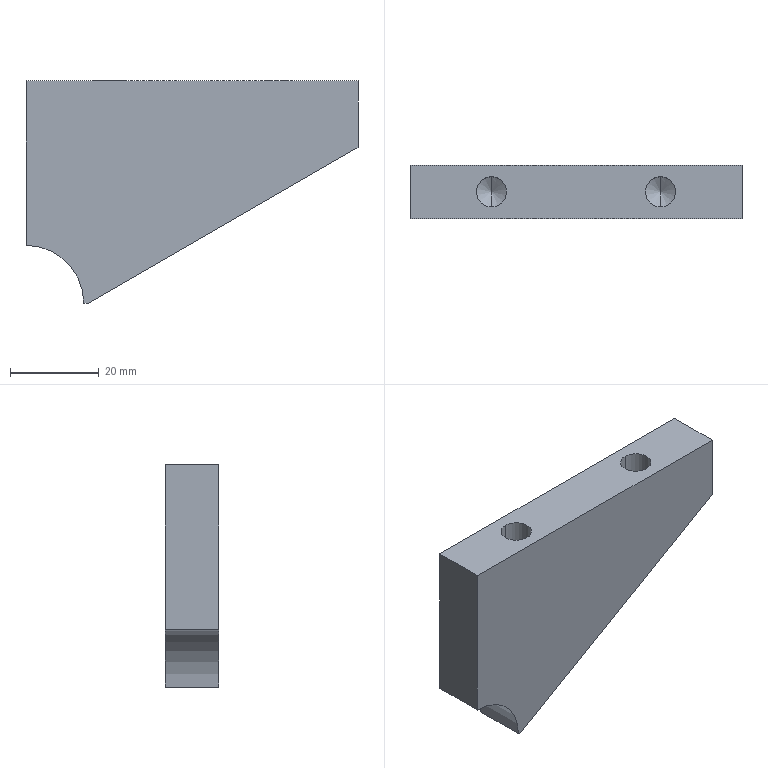Component | SolidWorks | StopBlock2-1 | 1 solid | 16 faces | box 74.62 x 12 x 50 mm | volume 28966 mm3 | plane 7 | cylinder 5 | cone 4 | commonest cylinder face diameters 6.8 x4 26 x1 | material Q235
build123d program:
from build123d import *

# Parameters (mm, degrees)
BOSS_EXTRUDE1_DEPTH   = 12
M8_TAPPED_HOLE1_D     = 6.8
M8_TAPPED_HOLE1_DEPTH = 19.75
M8_TAPPED_HOLE1_TIP   = 2.043
SKETCH4_R             = 13
CUT_EXTRUDE1_DEPTH    = 91.622


with BuildPart() as part:
    # Sketch1 → Boss-Extrude1 (new body)
    with BuildSketch(Plane.XY):
        Polygon((0, 0), (0, 50), (-14, 50), (-74.622, 15), (-74.622, 0), align=None)
    extrude(amount=BOSS_EXTRUDE1_DEPTH)

    # M8 Tapped Hole1
    with Locations(Plane(origin=(-56.311, 0, 6), x_dir=(0, 0, -1), z_dir=(0, -1, 0))):
        with Locations((0, 0), (0, 38)):
            Hole(M8_TAPPED_HOLE1_D / 2, depth=M8_TAPPED_HOLE1_DEPTH)
            with Locations((0, 0, -(M8_TAPPED_HOLE1_DEPTH + M8_TAPPED_HOLE1_TIP / 2))):  # 118° drill point
                Cone(0, M8_TAPPED_HOLE1_D / 2, M8_TAPPED_HOLE1_TIP, mode=Mode.SUBTRACT)

    # Sketch4 → Cut-Extrude1 (cut, through all)
    with BuildSketch(Plane.XY.offset(12)):
        with Locations((0, 50)):
            Circle(SKETCH4_R)
    extrude(amount=-CUT_EXTRUDE1_DEPTH, mode=Mode.SUBTRACT)


solid = part.part

# Placed as in the assembly
solid = solid.moved(Location((1.474, -118.917, -1190.957), (90, 0, -180)))
STEP:
#1=COLOUR_RGB('',0.7922,0.8196,0.9333);
#2=FILL_AREA_STYLE_COLOUR('',#1);
#3=FILL_AREA_STYLE('',(#2));
#4=SURFACE_STYLE_FILL_AREA(#3);
#5=SURFACE_SIDE_STYLE('',(#4));
#6=SURFACE_STYLE_USAGE(.BOTH.,#5);
#7=PRESENTATION_STYLE_ASSIGNMENT((#6));
#8=CARTESIAN_POINT('',(2.275,-5.052,-47.666));
#9=VERTEX_POINT('',#8);
#10=CARTESIAN_POINT('',(2.275,-4.784,-47.666));
#11=VERTEX_POINT('',#10);
#12=CARTESIAN_POINT('',(2.275,-4.918,-47.666));
#13=DIRECTION('',(0.,0.,1.));
#14=DIRECTION('',(0.,1.,0.));
#15=AXIS2_PLACEMENT_3D('',#12,#13,#14);
#16=CIRCLE('',#15,0.1339);
#17=EDGE_CURVE('',#9,#11,#16,.T.);
#18=ORIENTED_EDGE('',*,*,#17,.F.);
#19=CARTESIAN_POINT('',(2.275,-5.052,-46.888));
#20=VERTEX_POINT('',#19);
#21=CARTESIAN_POINT('',(2.275,-5.052,-46.888));
#22=DIRECTION('',(0.,0.,1.));
#23=VECTOR('',#22,39.37);
#24=LINE('',#21,#23);
#25=EDGE_CURVE('',#9,#20,#24,.T.);
#26=ORIENTED_EDGE('',*,*,#25,.T.);
#27=CARTESIAN_POINT('',(2.275,-4.784,-46.888));
#28=VERTEX_POINT('',#27);
#29=CARTESIAN_POINT('',(2.275,-4.918,-46.888));
#30=DIRECTION('',(0.,0.,1.));
#31=DIRECTION('',(0.,1.,0.));
#32=AXIS2_PLACEMENT_3D('',#29,#30,#31);
#33=CIRCLE('',#32,0.1339);
#34=EDGE_CURVE('',#20,#28,#33,.T.);
#35=ORIENTED_EDGE('',*,*,#34,.T.);
#36=CARTESIAN_POINT('',(2.275,-4.784,-46.888));
#37=DIRECTION('',(0.,0.,1.));
#38=VECTOR('',#37,39.37);
#39=LINE('',#36,#38);
#40=EDGE_CURVE('',#11,#28,#39,.T.);
#41=ORIENTED_EDGE('',*,*,#40,.F.);
#42=EDGE_LOOP('',(#18,#26,#35,#41));
#43=FACE_OUTER_BOUND('',#42,.T.);
#44=CARTESIAN_POINT('',(2.275,-4.918,-46.888));
#45=DIRECTION('',(0.,0.,1.));
#46=DIRECTION('',(0.,1.,0.));
#47=AXIS2_PLACEMENT_3D('',#44,#45,#46);
#48=CYLINDRICAL_SURFACE('',#47,0.1339);
#49=ADVANCED_FACE('',(#43),#48,.F.);
#50=CARTESIAN_POINT('',(2.275,-4.918,-47.746));
#51=VERTEX_POINT('',#50);
#52=CARTESIAN_POINT('',(2.275,-4.784,-47.666));
#53=DIRECTION('',(0.,0.8572,0.515));
#54=VECTOR('',#53,39.37);
#55=LINE('',#52,#54);
#56=EDGE_CURVE('',#51,#11,#55,.T.);
#57=ORIENTED_EDGE('',*,*,#56,.F.);
#58=CARTESIAN_POINT('',(2.275,-5.052,-47.666));
#59=DIRECTION('',(-0.,-0.8572,0.515));
#60=VECTOR('',#59,39.37);
#61=LINE('',#58,#60);
#62=EDGE_CURVE('',#51,#9,#61,.T.);
#63=ORIENTED_EDGE('',*,*,#62,.T.);
#64=ORIENTED_EDGE('',*,*,#17,.T.);
#65=EDGE_LOOP('',(#57,#63,#64));
#66=FACE_OUTER_BOUND('',#65,.T.);
#67=CARTESIAN_POINT('',(2.275,-4.918,-47.666));
#68=DIRECTION('',(0.,0.,1.));
#69=DIRECTION('',(0.,1.,0.));
#70=AXIS2_PLACEMENT_3D('',#67,#68,#69);
#71=CONICAL_SURFACE('',#70,0.1339,1.03);
#72=ADVANCED_FACE('',(#66),#71,.F.);
#73=CARTESIAN_POINT('',(0.7789,-5.052,-47.666));
#74=VERTEX_POINT('',#73);
#75=CARTESIAN_POINT('',(0.7789,-4.784,-47.666));
#76=VERTEX_POINT('',#75);
#77=CARTESIAN_POINT('',(0.7789,-4.918,-47.666));
#78=DIRECTION('',(0.,0.,1.));
#79=DIRECTION('',(0.,1.,0.));
#80=AXIS2_PLACEMENT_3D('',#77,#78,#79);
#81=CIRCLE('',#80,0.1339);
#82=EDGE_CURVE('',#74,#76,#81,.T.);
#83=ORIENTED_EDGE('',*,*,#82,.F.);
#84=CARTESIAN_POINT('',(0.7789,-5.052,-46.888));
#85=VERTEX_POINT('',#84);
#86=CARTESIAN_POINT('',(0.7789,-5.052,-46.888));
#87=DIRECTION('',(0.,0.,1.));
#88=VECTOR('',#87,39.37);
#89=LINE('',#86,#88);
#90=EDGE_CURVE('',#74,#85,#89,.T.);
#91=ORIENTED_EDGE('',*,*,#90,.T.);
#92=CARTESIAN_POINT('',(0.7789,-4.784,-46.888));
#93=VERTEX_POINT('',#92);
#94=CARTESIAN_POINT('',(0.7789,-4.918,-46.888));
#95=DIRECTION('',(0.,0.,1.));
#96=DIRECTION('',(0.,1.,0.));
#97=AXIS2_PLACEMENT_3D('',#94,#95,#96);
#98=CIRCLE('',#97,0.1339);
#99=EDGE_CURVE('',#85,#93,#98,.T.);
#100=ORIENTED_EDGE('',*,*,#99,.T.);
#101=CARTESIAN_POINT('',(0.7789,-4.784,-46.888));
#102=DIRECTION('',(0.,0.,1.));
#103=VECTOR('',#102,39.37);
#104=LINE('',#101,#103);
#105=EDGE_CURVE('',#76,#93,#104,.T.);
#106=ORIENTED_EDGE('',*,*,#105,.F.);
#107=EDGE_LOOP('',(#83,#91,#100,#106));
#108=FACE_OUTER_BOUND('',#107,.T.);
#109=CARTESIAN_POINT('',(0.7789,-4.918,-46.888));
#110=DIRECTION('',(0.,0.,1.));
#111=DIRECTION('',(0.,1.,0.));
#112=AXIS2_PLACEMENT_3D('',#109,#110,#111);
#113=CYLINDRICAL_SURFACE('',#112,0.1339);
#114=ADVANCED_FACE('',(#108),#113,.F.);
#115=CARTESIAN_POINT('',(0.7789,-4.918,-47.746));
#116=VERTEX_POINT('',#115);
#117=CARTESIAN_POINT('',(0.7789,-4.784,-47.666));
#118=DIRECTION('',(0.,0.8572,0.515));
#119=VECTOR('',#118,39.37);
#120=LINE('',#117,#119);
#121=EDGE_CURVE('',#116,#76,#120,.T.);
#122=ORIENTED_EDGE('',*,*,#121,.F.);
#123=CARTESIAN_POINT('',(0.7789,-5.052,-47.666));
#124=DIRECTION('',(-0.,-0.8572,0.515));
#125=VECTOR('',#124,39.37);
#126=LINE('',#123,#125);
#127=EDGE_CURVE('',#116,#74,#126,.T.);
#128=ORIENTED_EDGE('',*,*,#127,.T.);
#129=ORIENTED_EDGE('',*,*,#82,.T.);
#130=EDGE_LOOP('',(#122,#128,#129));
#131=FACE_OUTER_BOUND('',#130,.T.);
#132=CARTESIAN_POINT('',(0.7789,-4.918,-47.666));
#133=DIRECTION('',(0.,0.,1.));
#134=DIRECTION('',(0.,1.,0.));
#135=AXIS2_PLACEMENT_3D('',#132,#133,#134);
#136=CONICAL_SURFACE('',#135,0.1339,1.03);
#137=ADVANCED_FACE('',(#131),#136,.F.);
#138=CARTESIAN_POINT('',(2.275,-4.918,-46.888));
#139=DIRECTION('',(0.,0.,1.));
#140=DIRECTION('',(0.,1.,0.));
#141=AXIS2_PLACEMENT_3D('',#138,#139,#140);
#142=CIRCLE('',#141,0.1339);
#143=EDGE_CURVE('',#28,#20,#142,.T.);
#144=ORIENTED_EDGE('',*,*,#143,.F.);
#145=ORIENTED_EDGE('',*,*,#34,.F.);
#146=EDGE_LOOP('',(#144,#145));
#147=FACE_BOUND('',#146,.T.);
#148=CARTESIAN_POINT('',(0.7789,-4.918,-46.888));
#149=DIRECTION('',(0.,0.,1.));
#150=DIRECTION('',(0.,1.,0.));
#151=AXIS2_PLACEMENT_3D('',#148,#149,#150);
#152=CIRCLE('',#151,0.1339);
#153=EDGE_CURVE('',#93,#85,#152,.T.);
#154=ORIENTED_EDGE('',*,*,#153,.F.);
#155=ORIENTED_EDGE('',*,*,#99,.F.);
#156=EDGE_LOOP('',(#154,#155));
#157=FACE_BOUND('',#156,.T.);
#158=CARTESIAN_POINT('',(2.996,-4.682,-46.888));
#159=VERTEX_POINT('',#158);
#160=CARTESIAN_POINT('',(0.05803,-4.682,-46.888));
#161=VERTEX_POINT('',#160);
#162=CARTESIAN_POINT('',(2.996,-4.682,-46.888));
#163=DIRECTION('',(-1.,0.,0.));
#164=VECTOR('',#163,39.37);
#165=LINE('',#162,#164);
#166=EDGE_CURVE('',#159,#161,#165,.T.);
#167=ORIENTED_EDGE('',*,*,#166,.T.);
#168=CARTESIAN_POINT('',(0.05803,-5.154,-46.888));
#169=VERTEX_POINT('',#168);
#170=CARTESIAN_POINT('',(0.05803,-5.154,-46.888));
#171=DIRECTION('',(0.,1.,0.));
#172=VECTOR('',#171,39.37);
#173=LINE('',#170,#172);
#174=EDGE_CURVE('',#169,#161,#173,.T.);
#175=ORIENTED_EDGE('',*,*,#174,.F.);
#176=CARTESIAN_POINT('',(2.996,-5.154,-46.888));
#177=VERTEX_POINT('',#176);
#178=CARTESIAN_POINT('',(2.996,-5.154,-46.888));
#179=DIRECTION('',(-1.,0.,0.));
#180=VECTOR('',#179,39.37);
#181=LINE('',#178,#180);
#182=EDGE_CURVE('',#177,#169,#181,.T.);
#183=ORIENTED_EDGE('',*,*,#182,.F.);
#184=CARTESIAN_POINT('',(2.996,-5.154,-46.888));
#185=DIRECTION('',(0.,1.,0.));
#186=VECTOR('',#185,39.37);
#187=LINE('',#184,#186);
#188=EDGE_CURVE('',#177,#159,#187,.T.);
#189=ORIENTED_EDGE('',*,*,#188,.T.);
#190=EDGE_LOOP('',(#167,#175,#183,#189));
#191=FACE_OUTER_BOUND('',#190,.T.);
#192=CARTESIAN_POINT('',(2.996,-5.154,-46.888));
#193=DIRECTION('',(0.,0.,-1.));
#194=DIRECTION('',(0.,-1.,0.));
#195=AXIS2_PLACEMENT_3D('',#192,#193,#194);
#196=PLANE('',#195);
#197=ADVANCED_FACE('',(#147,#157,#191),#196,.F.);
#198=CARTESIAN_POINT('',(0.05803,-4.682,-48.345));
#199=VERTEX_POINT('',#198);
#200=CARTESIAN_POINT('',(0.05803,-4.682,-46.888));
#201=DIRECTION('',(0.,0.,-1.));
#202=VECTOR('',#201,39.37);
#203=LINE('',#200,#202);
#204=EDGE_CURVE('',#161,#199,#203,.T.);
#205=ORIENTED_EDGE('',*,*,#204,.T.);
#206=CARTESIAN_POINT('',(0.05803,-5.154,-48.345));
#207=VERTEX_POINT('',#206);
#208=CARTESIAN_POINT('',(0.05803,-4.682,-48.345));
#209=DIRECTION('',(0.,-1.,0.));
#210=VECTOR('',#209,39.37);
#211=LINE('',#208,#210);
#212=EDGE_CURVE('',#199,#207,#211,.T.);
#213=ORIENTED_EDGE('',*,*,#212,.T.);
#214=CARTESIAN_POINT('',(0.05803,-5.154,-46.888));
#215=DIRECTION('',(0.,0.,-1.));
#216=VECTOR('',#215,39.37);
#217=LINE('',#214,#216);
#218=EDGE_CURVE('',#169,#207,#217,.T.);
#219=ORIENTED_EDGE('',*,*,#218,.F.);
#220=ORIENTED_EDGE('',*,*,#174,.T.);
#221=EDGE_LOOP('',(#205,#213,#219,#220));
#222=FACE_OUTER_BOUND('',#221,.T.);
#223=CARTESIAN_POINT('',(0.05803,-5.154,-46.888));
#224=DIRECTION('',(1.,0.,0.));
#225=DIRECTION('',(0.,-1.,0.));
#226=AXIS2_PLACEMENT_3D('',#223,#224,#225);
#227=PLANE('',#226);
#228=ADVANCED_FACE('',(#222),#227,.F.);
#229=CARTESIAN_POINT('',(0.5698,-5.154,-48.857));
#230=VERTEX_POINT('',#229);
#231=CARTESIAN_POINT('',(0.6092,-5.154,-48.857));
#232=VERTEX_POINT('',#231);
#233=CARTESIAN_POINT('',(0.05803,-5.154,-48.857));
#234=DIRECTION('',(1.,0.,0.));
#235=VECTOR('',#234,39.37);
#236=LINE('',#233,#235);
#237=EDGE_CURVE('',#230,#232,#236,.T.);
#238=ORIENTED_EDGE('',*,*,#237,.F.);
#239=CARTESIAN_POINT('',(0.5698,-4.682,-48.857));
#240=VERTEX_POINT('',#239);
#241=CARTESIAN_POINT('',(0.5698,-4.682,-48.857));
#242=DIRECTION('',(0.,1.,0.));
#243=VECTOR('',#242,39.37);
#244=LINE('',#241,#243);
#245=EDGE_CURVE('',#230,#240,#244,.T.);
#246=ORIENTED_EDGE('',*,*,#245,.T.);
#247=CARTESIAN_POINT('',(0.6092,-4.682,-48.857));
#248=VERTEX_POINT('',#247);
#249=CARTESIAN_POINT('',(0.05803,-4.682,-48.857));
#250=DIRECTION('',(1.,0.,0.));
#251=VECTOR('',#250,39.37);
#252=LINE('',#249,#251);
#253=EDGE_CURVE('',#240,#248,#252,.T.);
#254=ORIENTED_EDGE('',*,*,#253,.T.);
#255=CARTESIAN_POINT('',(0.6092,-5.154,-48.857));
#256=DIRECTION('',(0.,1.,0.));
#257=VECTOR('',#256,39.37);
#258=LINE('',#255,#257);
#259=EDGE_CURVE('',#232,#248,#258,.T.);
#260=ORIENTED_EDGE('',*,*,#259,.F.);
#261=EDGE_LOOP('',(#238,#246,#254,#260));
#262=FACE_OUTER_BOUND('',#261,.T.);
#263=CARTESIAN_POINT('',(0.05803,-5.154,-48.857));
#264=DIRECTION('',(0.,0.,1.));
#265=DIRECTION('',(0.,1.,0.));
#266=AXIS2_PLACEMENT_3D('',#263,#264,#265);
#267=PLANE('',#266);
#268=ADVANCED_FACE('',(#262),#267,.F.);
#269=CARTESIAN_POINT('',(2.996,-4.682,-47.479));
#270=VERTEX_POINT('',#269);
#271=CARTESIAN_POINT('',(2.996,-4.682,-47.479));
#272=DIRECTION('',(0.866,0.,0.5));
#273=VECTOR('',#272,39.37);
#274=LINE('',#271,#273);
#275=EDGE_CURVE('',#248,#270,#274,.T.);
#276=ORIENTED_EDGE('',*,*,#275,.T.);
#277=CARTESIAN_POINT('',(2.996,-5.154,-47.479));
#278=VERTEX_POINT('',#277);
#279=CARTESIAN_POINT('',(2.996,-5.154,-47.479));
#280=DIRECTION('',(0.,1.,0.));
#281=VECTOR('',#280,39.37);
#282=LINE('',#279,#281);
#283=EDGE_CURVE('',#278,#270,#282,.T.);
#284=ORIENTED_EDGE('',*,*,#283,.F.);
#285=CARTESIAN_POINT('',(2.996,-5.154,-47.479));
#286=DIRECTION('',(0.866,0.,0.5));
#287=VECTOR('',#286,39.37);
#288=LINE('',#285,#287);
#289=EDGE_CURVE('',#232,#278,#288,.T.);
#290=ORIENTED_EDGE('',*,*,#289,.F.);
#291=ORIENTED_EDGE('',*,*,#259,.T.);
#292=EDGE_LOOP('',(#276,#284,#290,#291));
#293=FACE_OUTER_BOUND('',#292,.T.);
#294=CARTESIAN_POINT('',(2.996,-5.154,-47.479));
#295=DIRECTION('',(-0.5,0.,0.866));
#296=DIRECTION('',(-0.866,0.,-0.5));
#297=AXIS2_PLACEMENT_3D('',#294,#295,#296);
#298=PLANE('',#297);
#299=ADVANCED_FACE('',(#293),#298,.F.);
#300=CARTESIAN_POINT('',(2.996,-4.682,-46.888));
#301=DIRECTION('',(0.,0.,1.));
#302=VECTOR('',#301,39.37);
#303=LINE('',#300,#302);
#304=EDGE_CURVE('',#270,#159,#303,.T.);
#305=ORIENTED_EDGE('',*,*,#304,.T.);
#306=ORIENTED_EDGE('',*,*,#188,.F.);
#307=CARTESIAN_POINT('',(2.996,-5.154,-46.888));
#308=DIRECTION('',(0.,0.,1.));
#309=VECTOR('',#308,39.37);
#310=LINE('',#307,#309);
#311=EDGE_CURVE('',#278,#177,#310,.T.);
#312=ORIENTED_EDGE('',*,*,#311,.F.);
#313=ORIENTED_EDGE('',*,*,#283,.T.);
#314=EDGE_LOOP('',(#305,#306,#312,#313));
#315=FACE_OUTER_BOUND('',#314,.T.);
#316=CARTESIAN_POINT('',(2.996,-5.154,-46.888));
#317=DIRECTION('',(-1.,0.,0.));
#318=DIRECTION('',(0.,1.,0.));
#319=AXIS2_PLACEMENT_3D('',#316,#317,#318);
#320=PLANE('',#319);
#321=ADVANCED_FACE('',(#315),#320,.F.);
#322=CARTESIAN_POINT('',(0.05803,-5.154,-48.857));
#323=DIRECTION('',(0.,-1.,0.));
#324=DIRECTION('',(-1.,0.,0.));
#325=AXIS2_PLACEMENT_3D('',#322,#323,#324);
#326=CIRCLE('',#325,0.5118);
#327=EDGE_CURVE('',#230,#207,#326,.T.);
#328=ORIENTED_EDGE('',*,*,#327,.F.);
#329=ORIENTED_EDGE('',*,*,#237,.T.);
#330=ORIENTED_EDGE('',*,*,#289,.T.);
#331=ORIENTED_EDGE('',*,*,#311,.T.);
#332=ORIENTED_EDGE('',*,*,#182,.T.);
#333=ORIENTED_EDGE('',*,*,#218,.T.);
#334=EDGE_LOOP('',(#328,#329,#330,#331,#332,#333));
#335=FACE_OUTER_BOUND('',#334,.T.);
#336=CARTESIAN_POINT('',(0.05803,-5.154,-46.888));
#337=DIRECTION('',(0.,-1.,0.));
#338=DIRECTION('',(-1.,0.,0.));
#339=AXIS2_PLACEMENT_3D('',#336,#337,#338);
#340=PLANE('',#339);
#341=ADVANCED_FACE('',(#335),#340,.T.);
#342=ORIENTED_EDGE('',*,*,#253,.F.);
#343=CARTESIAN_POINT('',(0.05803,-4.682,-48.857));
#344=DIRECTION('',(0.,-1.,0.));
#345=DIRECTION('',(-1.,0.,0.));
#346=AXIS2_PLACEMENT_3D('',#343,#344,#345);
#347=CIRCLE('',#346,0.5118);
#348=EDGE_CURVE('',#240,#199,#347,.T.);
#349=ORIENTED_EDGE('',*,*,#348,.T.);
#350=ORIENTED_EDGE('',*,*,#204,.F.);
#351=ORIENTED_EDGE('',*,*,#166,.F.);
#352=ORIENTED_EDGE('',*,*,#304,.F.);
#353=ORIENTED_EDGE('',*,*,#275,.F.);
#354=EDGE_LOOP('',(#342,#349,#350,#351,#352,#353));
#355=FACE_OUTER_BOUND('',#354,.T.);
#356=CARTESIAN_POINT('',(0.05803,-4.682,-46.888));
#357=DIRECTION('',(0.,-1.,0.));
#358=DIRECTION('',(-1.,0.,0.));
#359=AXIS2_PLACEMENT_3D('',#356,#357,#358);
#360=PLANE('',#359);
#361=ADVANCED_FACE('',(#355),#360,.F.);
#362=ORIENTED_EDGE('',*,*,#127,.F.);
#363=ORIENTED_EDGE('',*,*,#121,.T.);
#364=CARTESIAN_POINT('',(0.7789,-4.918,-47.666));
#365=DIRECTION('',(0.,0.,1.));
#366=DIRECTION('',(0.,1.,0.));
#367=AXIS2_PLACEMENT_3D('',#364,#365,#366);
#368=CIRCLE('',#367,0.1339);
#369=EDGE_CURVE('',#76,#74,#368,.T.);
#370=ORIENTED_EDGE('',*,*,#369,.T.);
#371=EDGE_LOOP('',(#362,#363,#370));
#372=FACE_OUTER_BOUND('',#371,.T.);
#373=CARTESIAN_POINT('',(0.7789,-4.918,-47.666));
#374=DIRECTION('',(0.,0.,1.));
#375=DIRECTION('',(0.,1.,0.));
#376=AXIS2_PLACEMENT_3D('',#373,#374,#375);
#377=CONICAL_SURFACE('',#376,0.1339,1.03);
#378=ADVANCED_FACE('',(#372),#377,.F.);
#379=ORIENTED_EDGE('',*,*,#90,.F.);
#380=ORIENTED_EDGE('',*,*,#369,.F.);
#381=ORIENTED_EDGE('',*,*,#105,.T.);
#382=ORIENTED_EDGE('',*,*,#153,.T.);
#383=EDGE_LOOP('',(#379,#380,#381,#382));
#384=FACE_OUTER_BOUND('',#383,.T.);
#385=CARTESIAN_POINT('',(0.7789,-4.918,-46.888));
#386=DIRECTION('',(0.,0.,1.));
#387=DIRECTION('',(0.,1.,0.));
#388=AXIS2_PLACEMENT_3D('',#385,#386,#387);
#389=CYLINDRICAL_SURFACE('',#388,0.1339);
#390=ADVANCED_FACE('',(#384),#389,.F.);
#391=ORIENTED_EDGE('',*,*,#62,.F.);
#392=ORIENTED_EDGE('',*,*,#56,.T.);
#393=CARTESIAN_POINT('',(2.275,-4.918,-47.666));
#394=DIRECTION('',(0.,0.,1.));
#395=DIRECTION('',(0.,1.,0.));
#396=AXIS2_PLACEMENT_3D('',#393,#394,#395);
#397=CIRCLE('',#396,0.1339);
#398=EDGE_CURVE('',#11,#9,#397,.T.);
#399=ORIENTED_EDGE('',*,*,#398,.T.);
#400=EDGE_LOOP('',(#391,#392,#399));
#401=FACE_OUTER_BOUND('',#400,.T.);
#402=CARTESIAN_POINT('',(2.275,-4.918,-47.666));
#403=DIRECTION('',(0.,0.,1.));
#404=DIRECTION('',(0.,1.,0.));
#405=AXIS2_PLACEMENT_3D('',#402,#403,#404);
#406=CONICAL_SURFACE('',#405,0.1339,1.03);
#407=ADVANCED_FACE('',(#401),#406,.F.);
#408=ORIENTED_EDGE('',*,*,#25,.F.);
#409=ORIENTED_EDGE('',*,*,#398,.F.);
#410=ORIENTED_EDGE('',*,*,#40,.T.);
#411=ORIENTED_EDGE('',*,*,#143,.T.);
#412=EDGE_LOOP('',(#408,#409,#410,#411));
#413=FACE_OUTER_BOUND('',#412,.T.);
#414=CARTESIAN_POINT('',(2.275,-4.918,-46.888));
#415=DIRECTION('',(0.,0.,1.));
#416=DIRECTION('',(0.,1.,0.));
#417=AXIS2_PLACEMENT_3D('',#414,#415,#416);
#418=CYLINDRICAL_SURFACE('',#417,0.1339);
#419=ADVANCED_FACE('',(#413),#418,.F.);
#420=ORIENTED_EDGE('',*,*,#348,.F.);
#421=ORIENTED_EDGE('',*,*,#245,.F.);
#422=ORIENTED_EDGE('',*,*,#327,.T.);
#423=ORIENTED_EDGE('',*,*,#212,.F.);
#424=EDGE_LOOP('',(#420,#421,#422,#423));
#425=FACE_OUTER_BOUND('',#424,.T.);
#426=CARTESIAN_POINT('',(0.05803,-4.682,-48.857));
#427=DIRECTION('',(0.,-1.,0.));
#428=DIRECTION('',(-1.,0.,0.));
#429=AXIS2_PLACEMENT_3D('',#426,#427,#428);
#430=CYLINDRICAL_SURFACE('',#429,0.5118);
#431=ADVANCED_FACE('',(#425),#430,.F.);
#432=CLOSED_SHELL('',(#49,#72,#114,#137,#197,#228,#268,#299,#321,#341,#361,#378,#390,#407,#419,#431));
#433=MANIFOLD_SOLID_BREP('',#432);
#434=STYLED_ITEM('',(#7),#433);
#435=(LENGTH_UNIT()NAMED_UNIT(*)SI_UNIT($,.METRE.));
#436=LENGTH_MEASURE_WITH_UNIT(LENGTH_MEASURE(0.0254),#435);
#437=DIMENSIONAL_EXPONENTS(1.,0.,0.,0.,0.,0.,0.);
#438=(CONVERSION_BASED_UNIT('',#436)LENGTH_UNIT()NAMED_UNIT(#437));
#439=UNCERTAINTY_MEASURE_WITH_UNIT(LENGTH_MEASURE(0.00001),#438,'','');
#440=(NAMED_UNIT(*)PLANE_ANGLE_UNIT()SI_UNIT($,.RADIAN.));
#441=(NAMED_UNIT(*)SI_UNIT($,.STERADIAN.)SOLID_ANGLE_UNIT());
#442=(GEOMETRIC_REPRESENTATION_CONTEXT(3)GLOBAL_UNCERTAINTY_ASSIGNED_CONTEXT((#439))GLOBAL_UNIT_ASSIGNED_CONTEXT((#438,#440,#441))REPRESENTATION_CONTEXT('',''));
#443=MECHANICAL_DESIGN_GEOMETRIC_PRESENTATION_REPRESENTATION('',(#434),#442);
#444=CARTESIAN_POINT('',(0.,0.,0.));
#445=DIRECTION('',(0.,0.,1.));
#446=DIRECTION('',(1.,0.,0.));
#447=AXIS2_PLACEMENT_3D('',#444,#445,#446);
#448=(LENGTH_UNIT()NAMED_UNIT(*)SI_UNIT($,.METRE.));
#449=LENGTH_MEASURE_WITH_UNIT(LENGTH_MEASURE(0.0254),#448);
#450=DIMENSIONAL_EXPONENTS(1.,0.,0.,0.,0.,0.,0.);
#451=(CONVERSION_BASED_UNIT('',#449)LENGTH_UNIT()NAMED_UNIT(#450));
#452=UNCERTAINTY_MEASURE_WITH_UNIT(LENGTH_MEASURE(0.00001),#451,'','');
#453=(NAMED_UNIT(*)PLANE_ANGLE_UNIT()SI_UNIT($,.RADIAN.));
#454=(NAMED_UNIT(*)SI_UNIT($,.STERADIAN.)SOLID_ANGLE_UNIT());
#455=(GEOMETRIC_REPRESENTATION_CONTEXT(3)GLOBAL_UNCERTAINTY_ASSIGNED_CONTEXT((#452))GLOBAL_UNIT_ASSIGNED_CONTEXT((#451,#453,#454))REPRESENTATION_CONTEXT('',''));
#456=ADVANCED_BREP_SHAPE_REPRESENTATION('',(#433,#447),#455);
#457=PRESENTATION_LAYER_ASSIGNMENT('','',(#434));